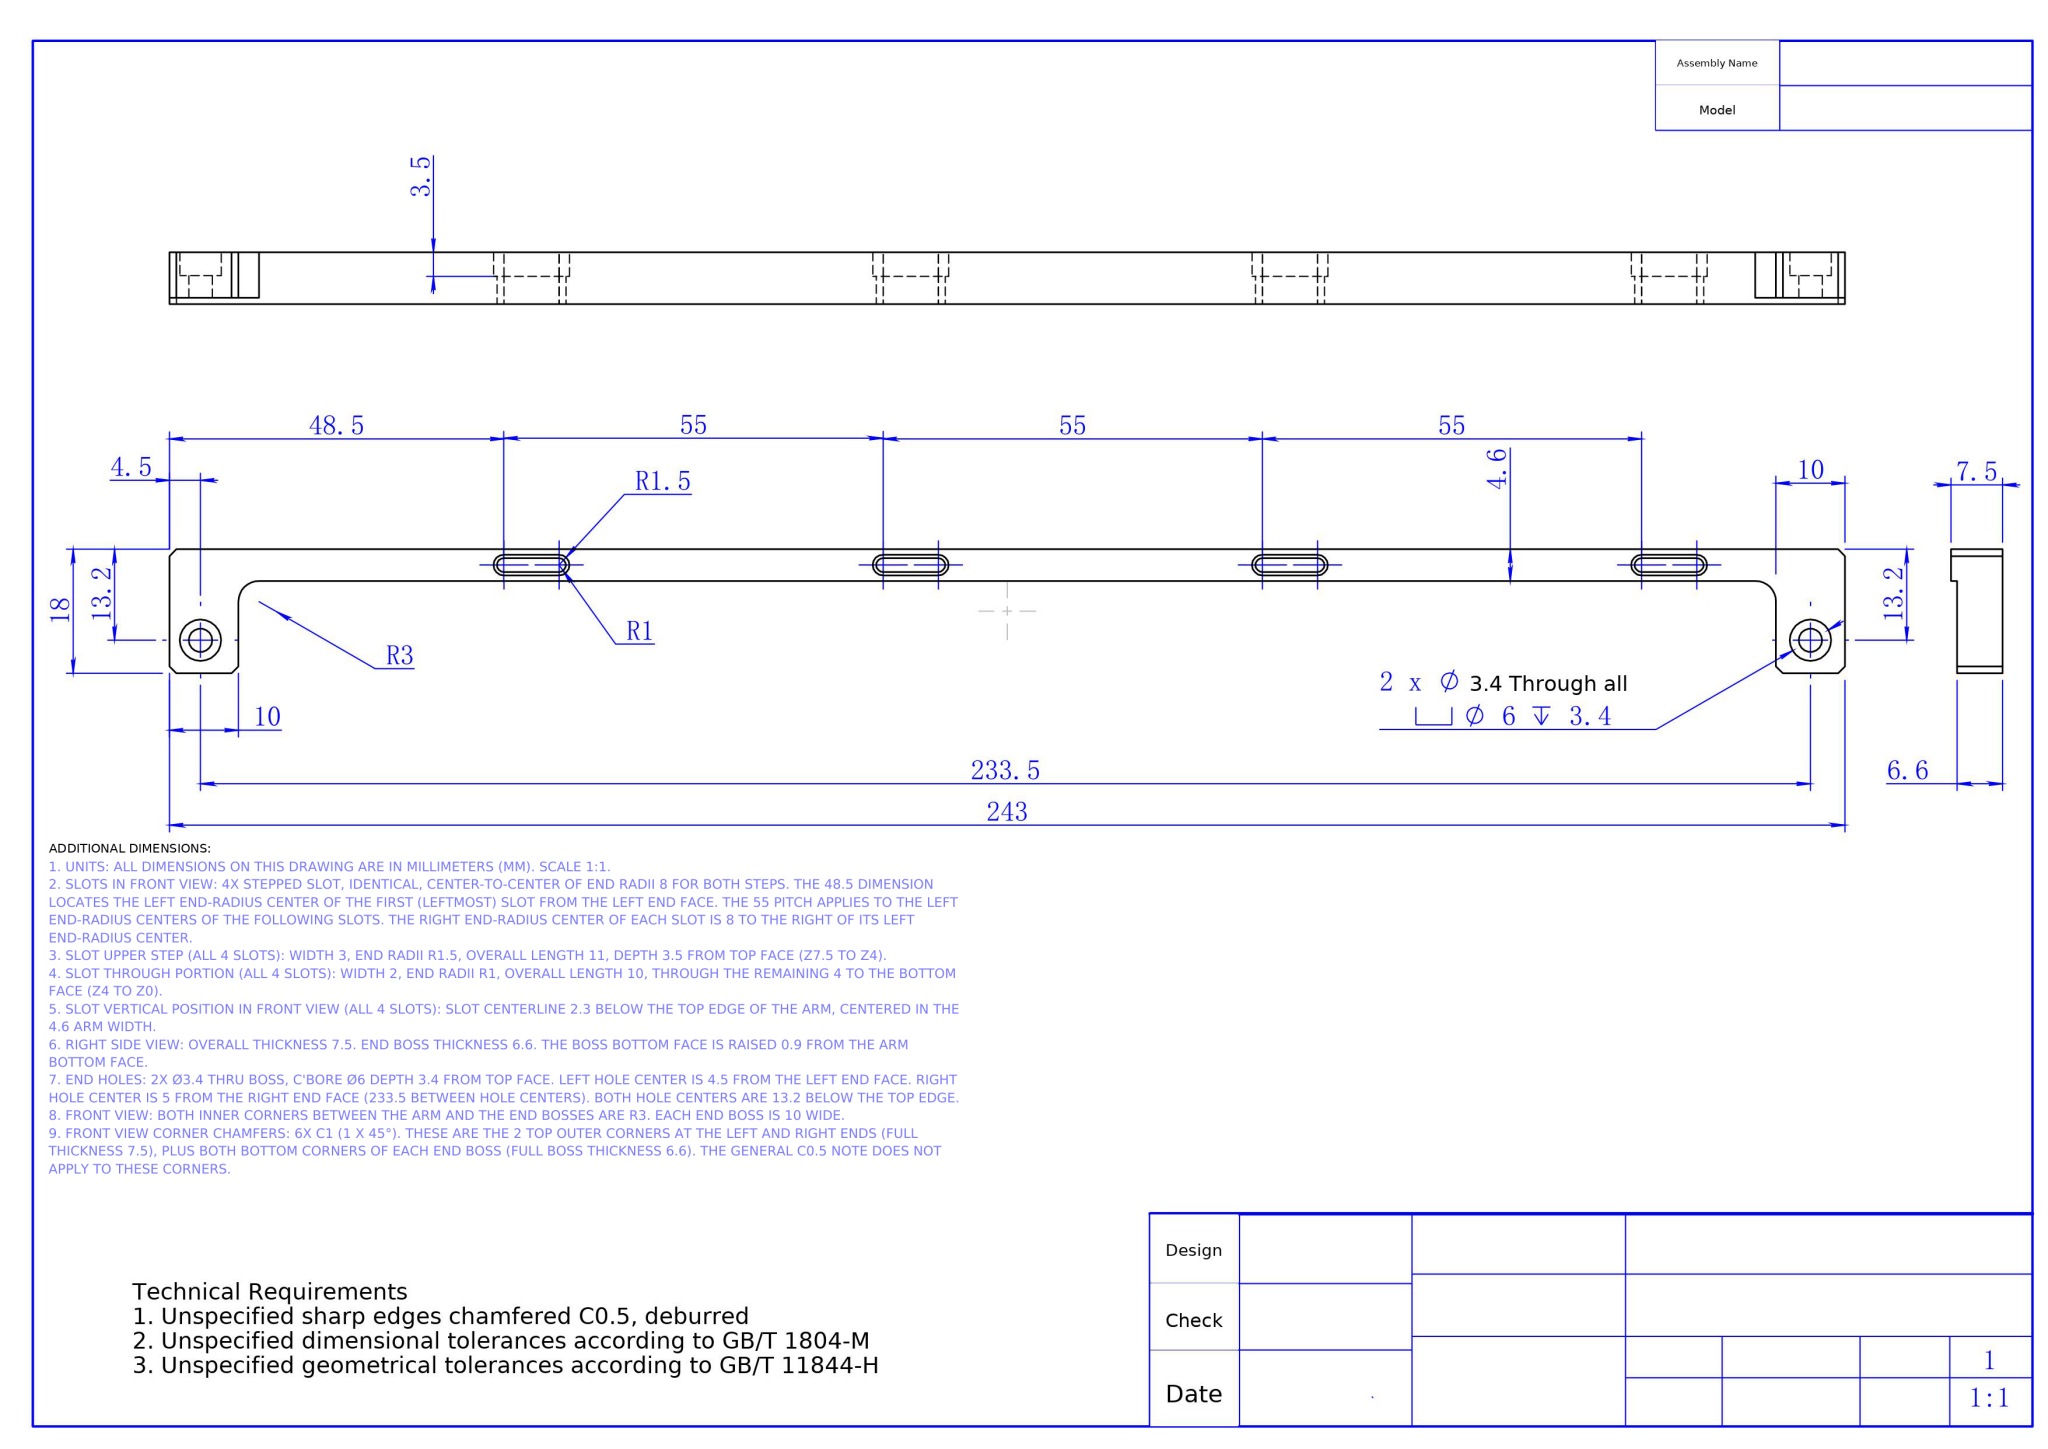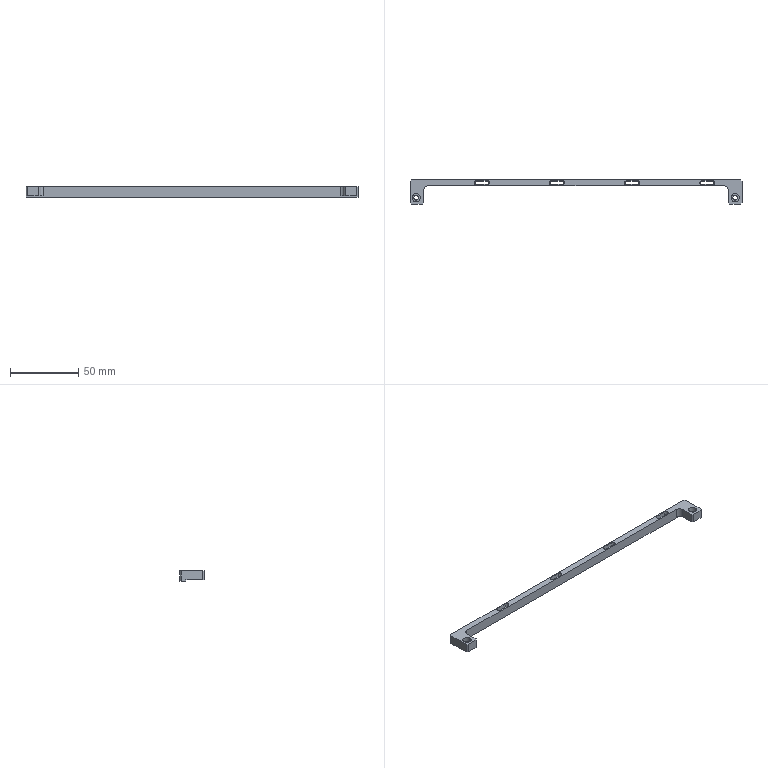Part | NX | mm | 1 solid | 74 faces | box 243 x 18 x 7.5 mm | volume 9165 mm3 | plane 40 | cylinder 34 | commonest cylinder face diameters 3 x12 2 x12 6 x6 3.4 x4